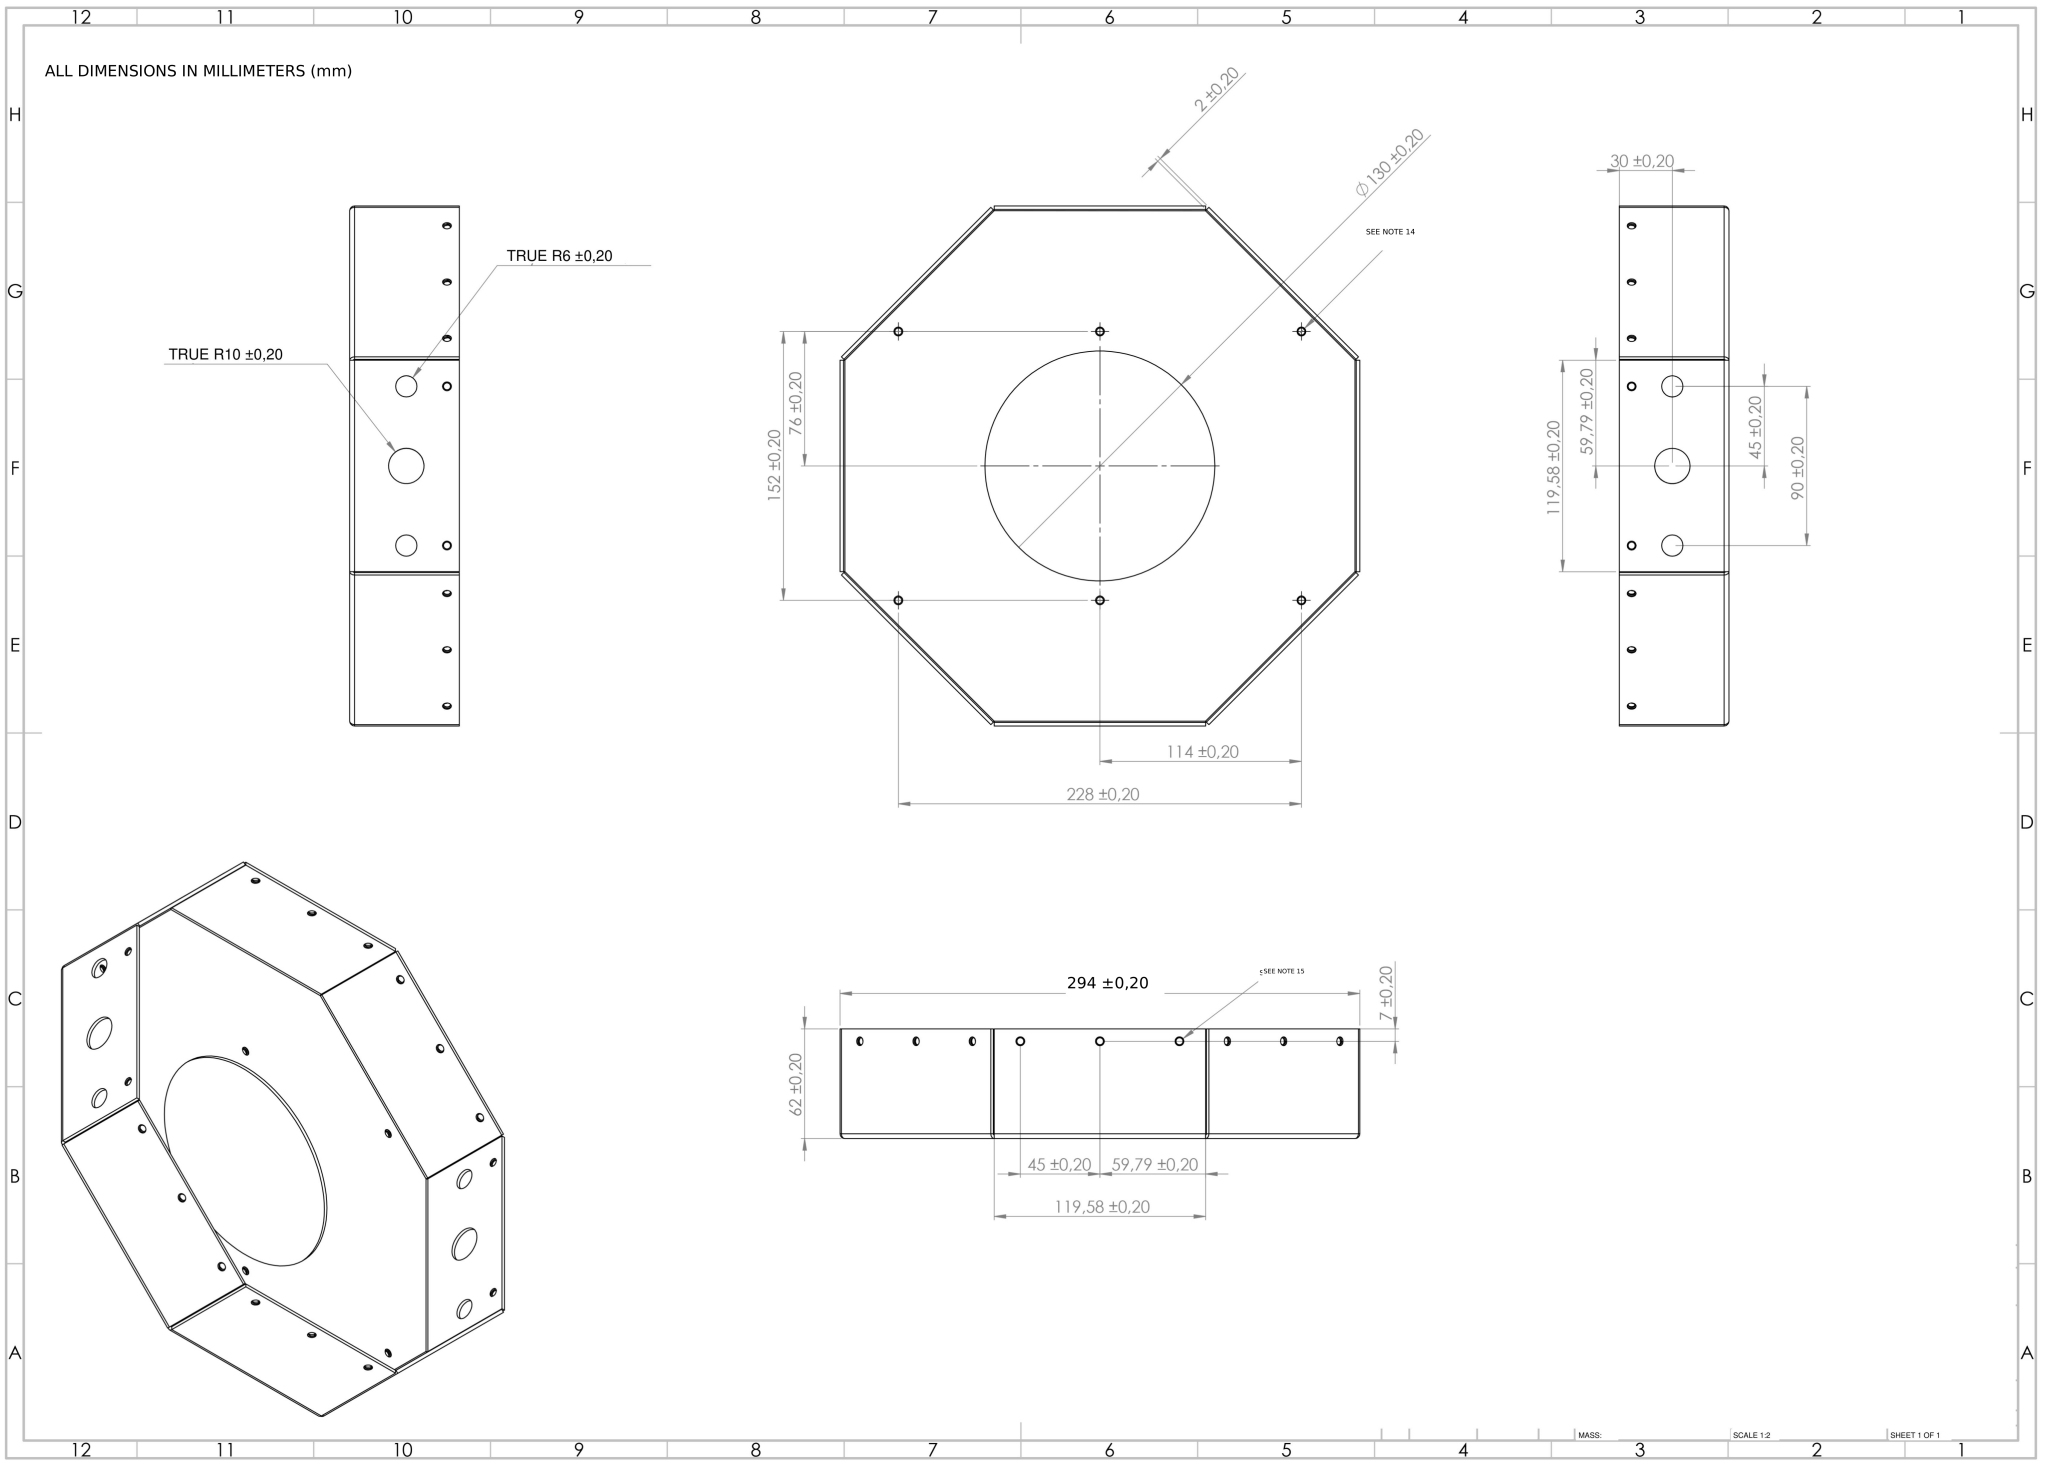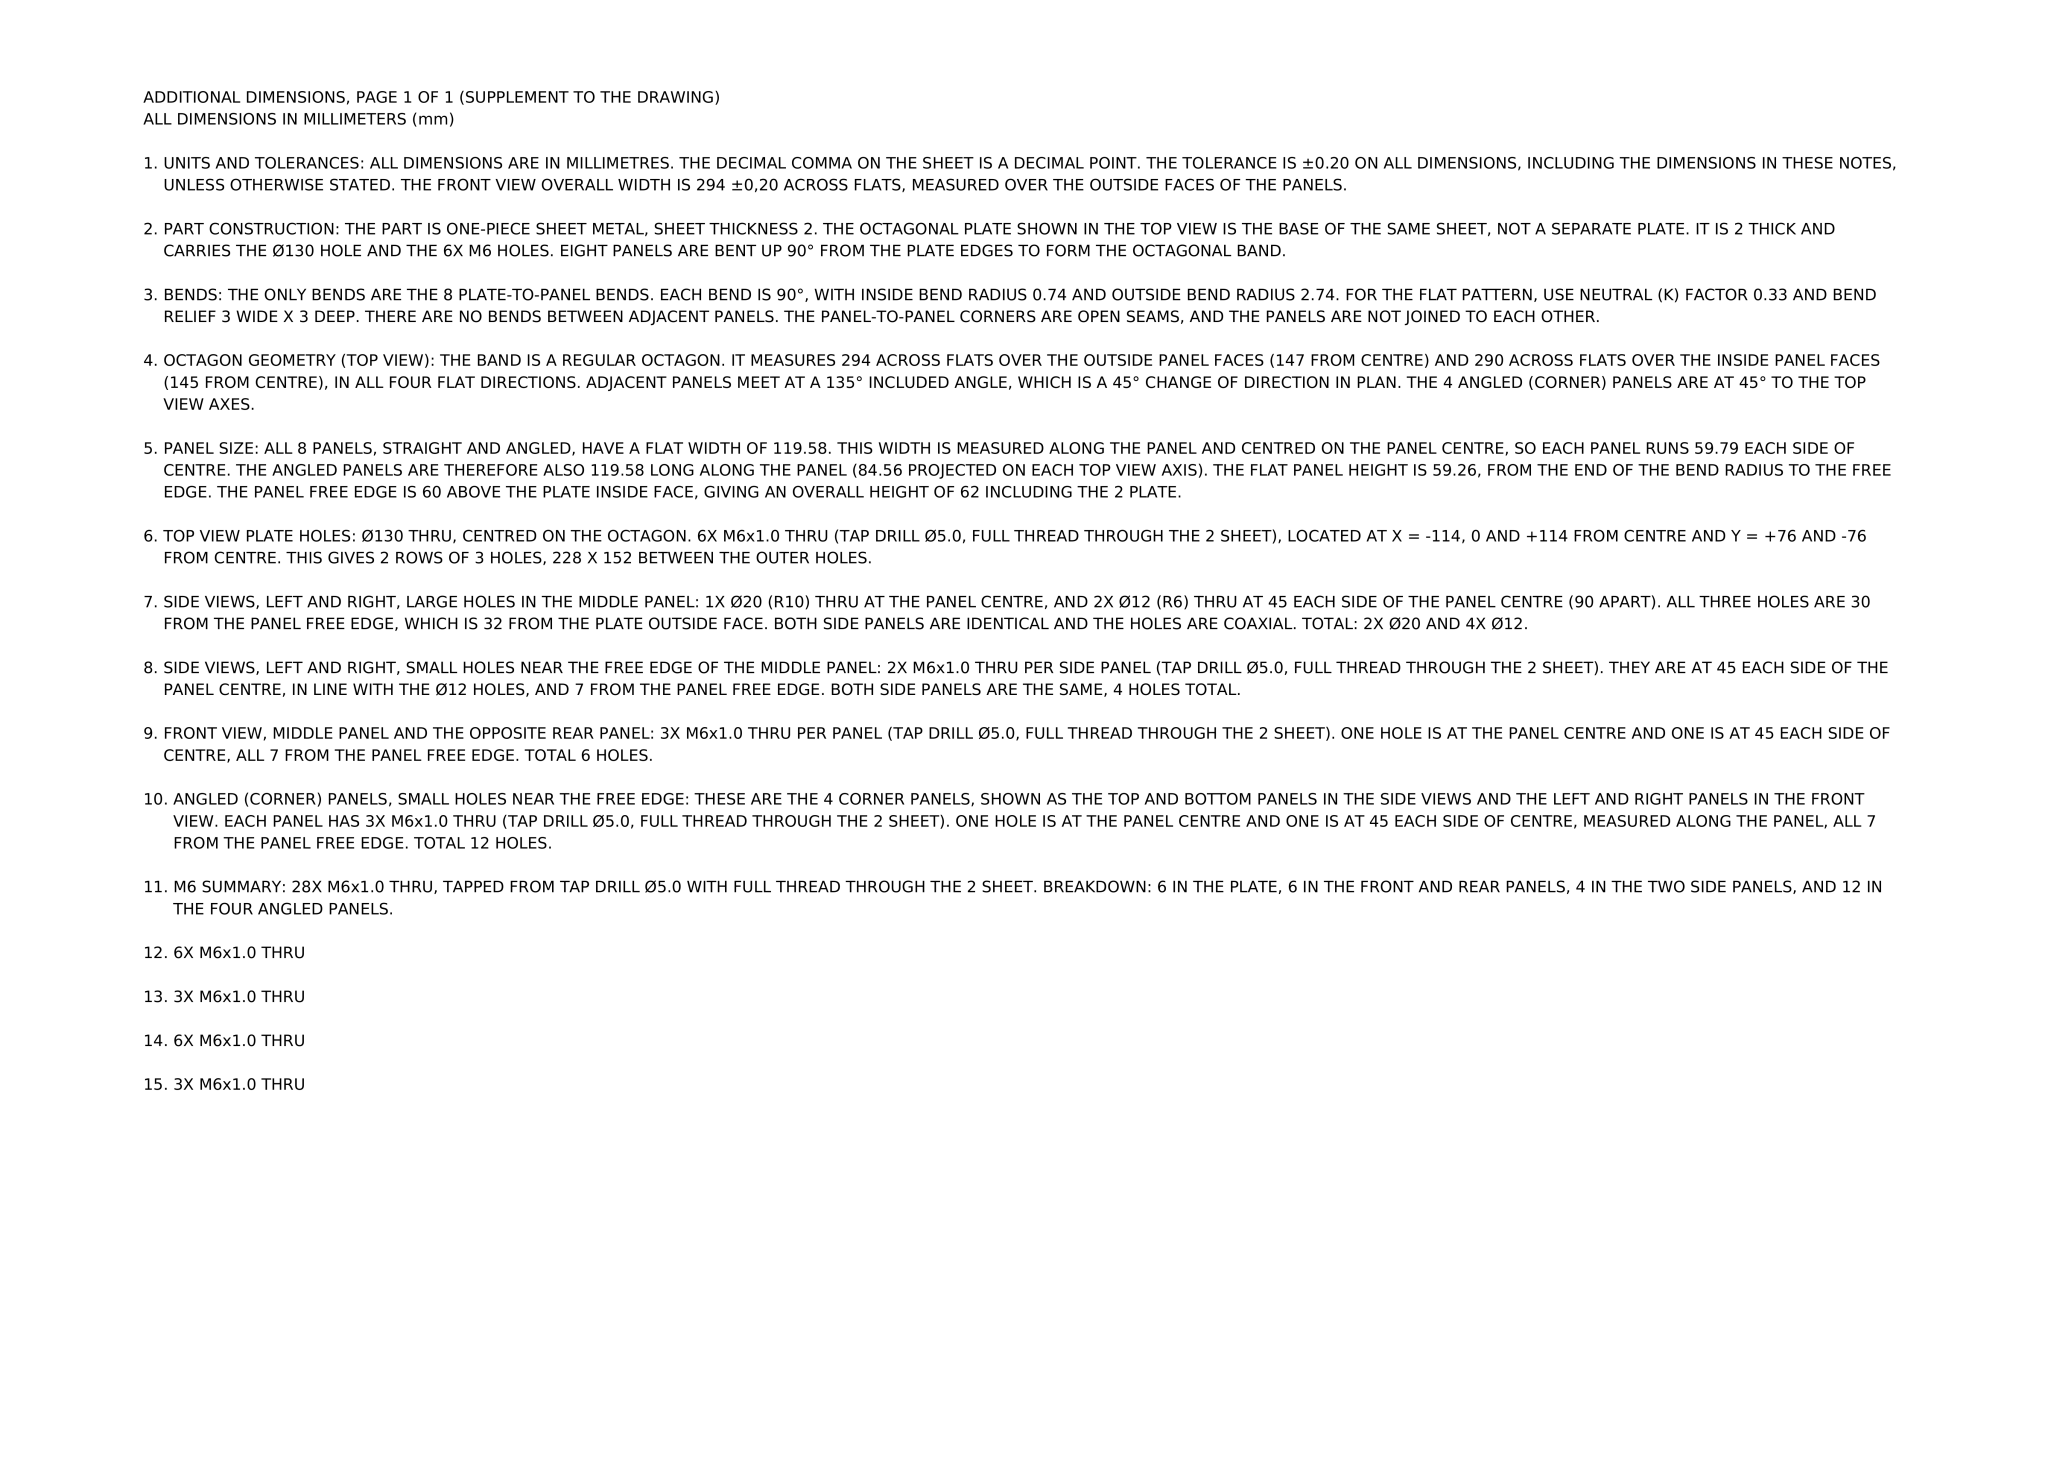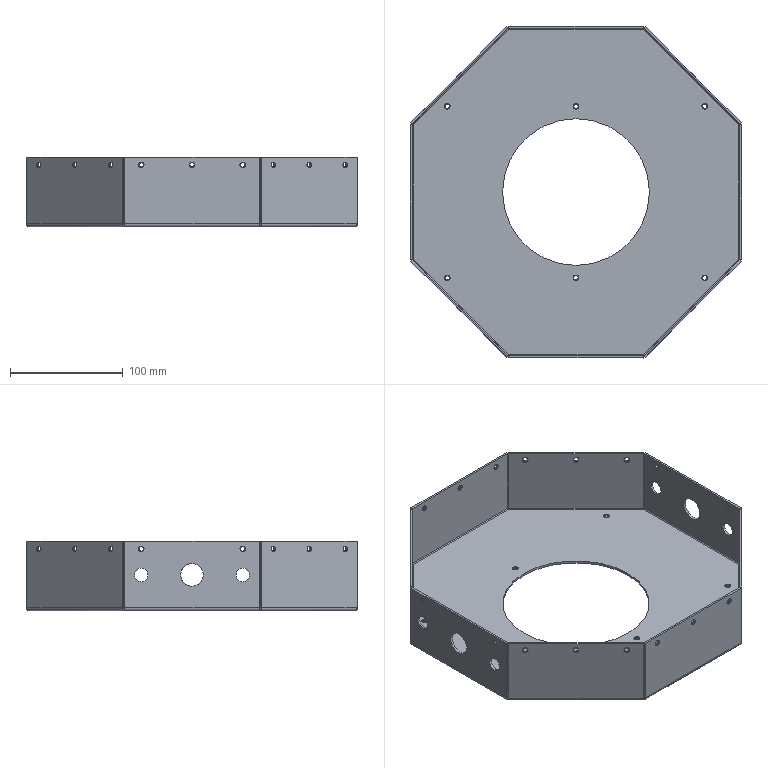Part | NX | mm | 1 solid | 340 faces | box 294.01 x 294.01 x 62 mm | volume 226850 mm3 | cylinder 142 | spline 100 | plane 98 | commonest cylinder face diameters 5 x112 12 x8 5.473 x8 1.473 x8 20 x4 130 x2